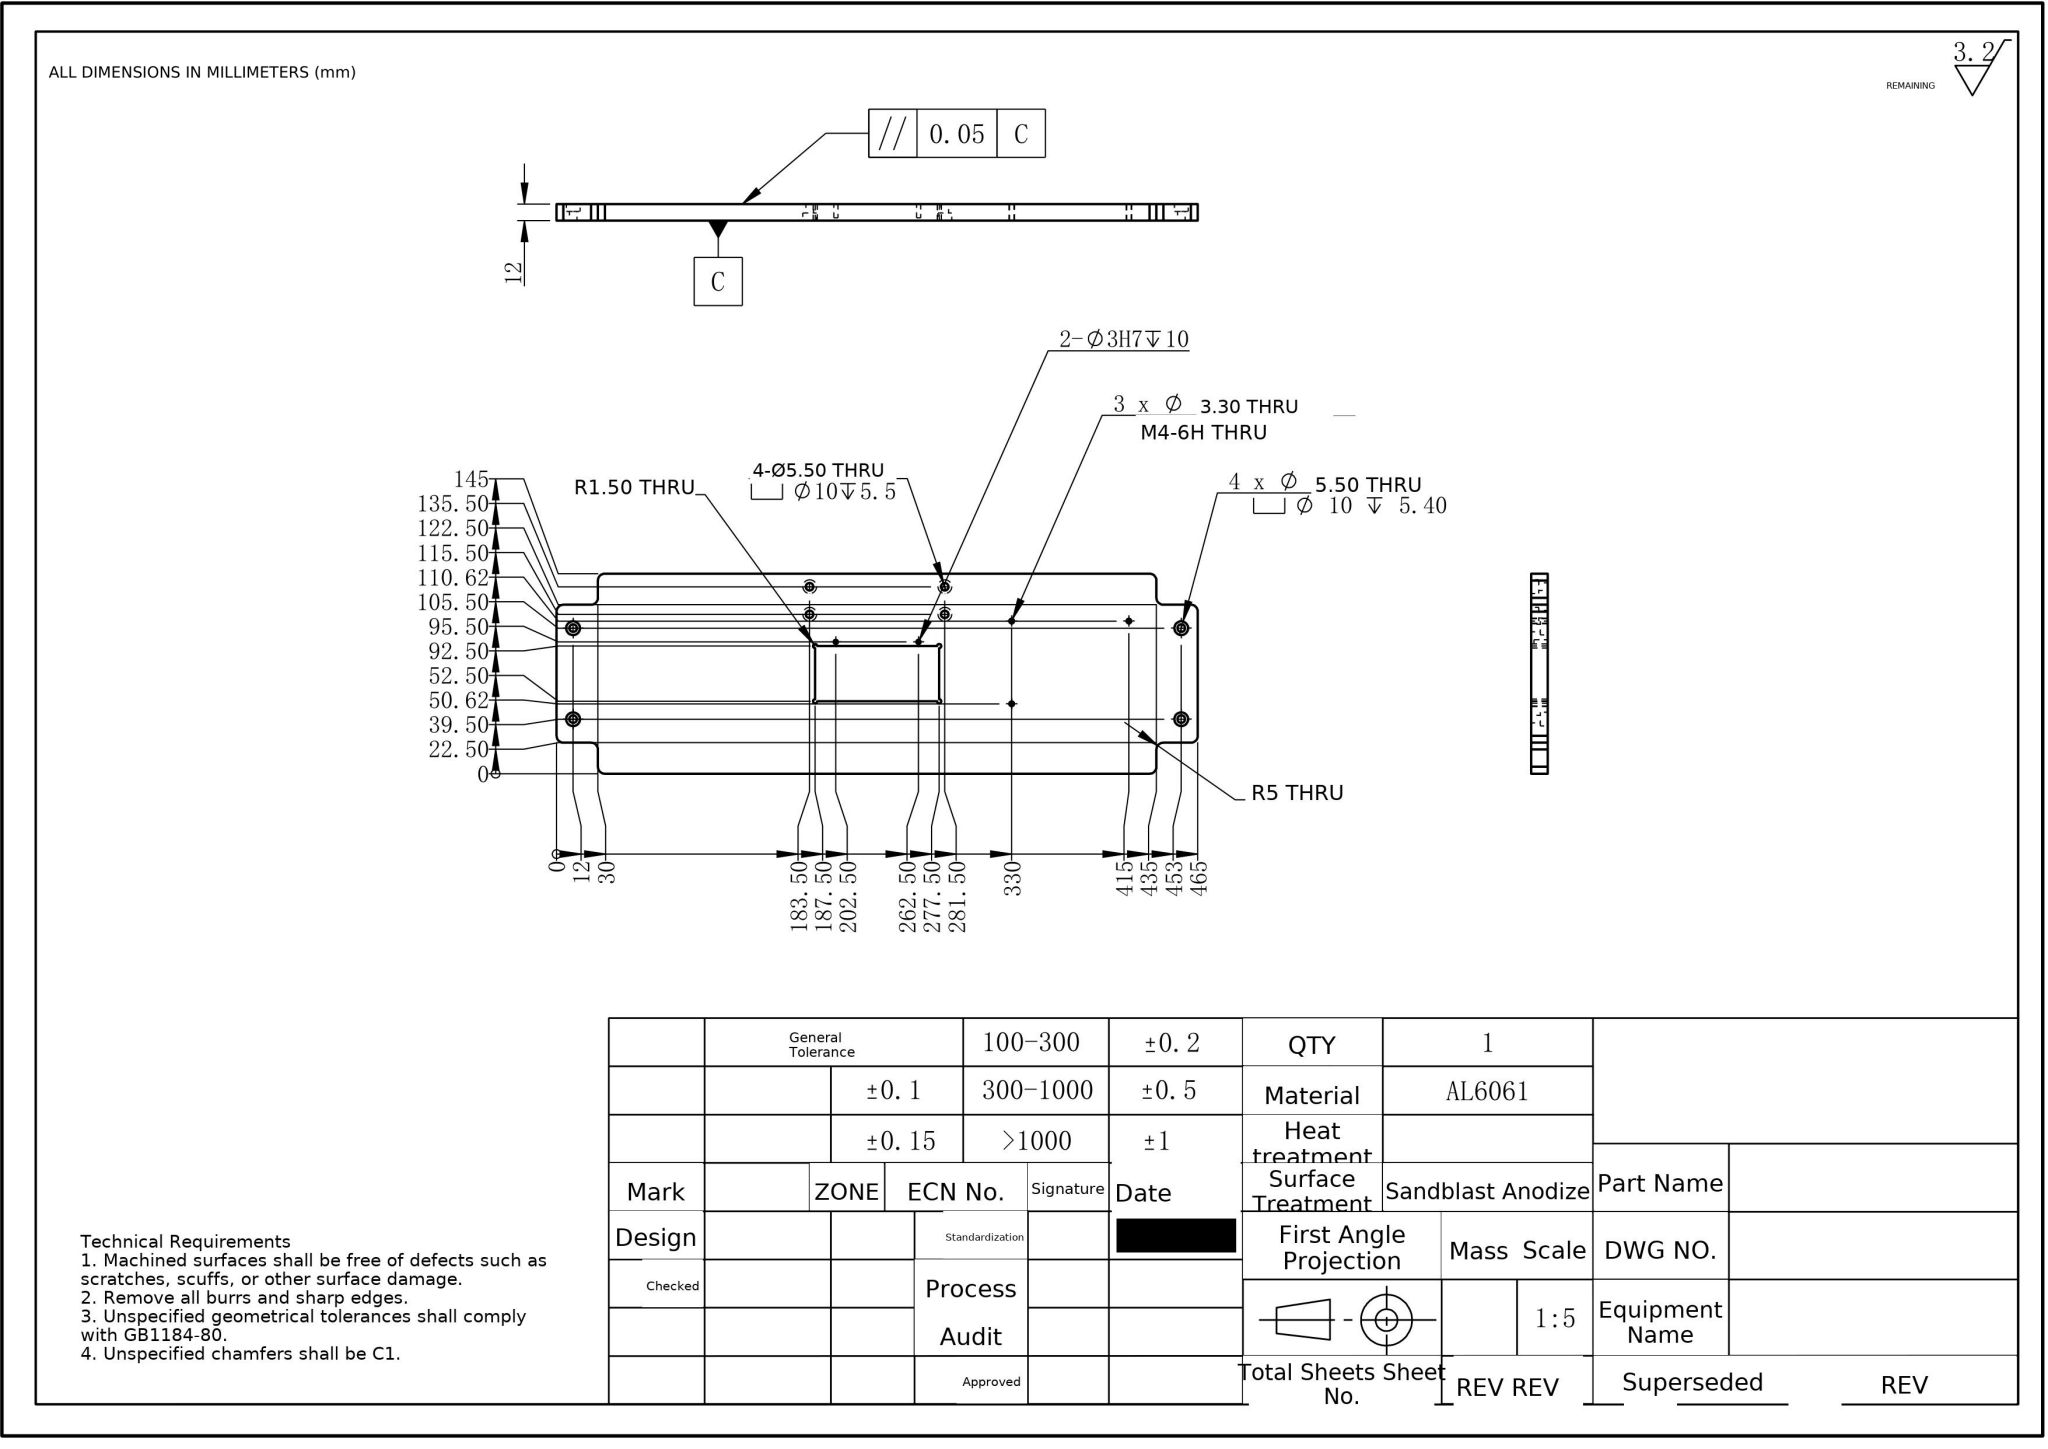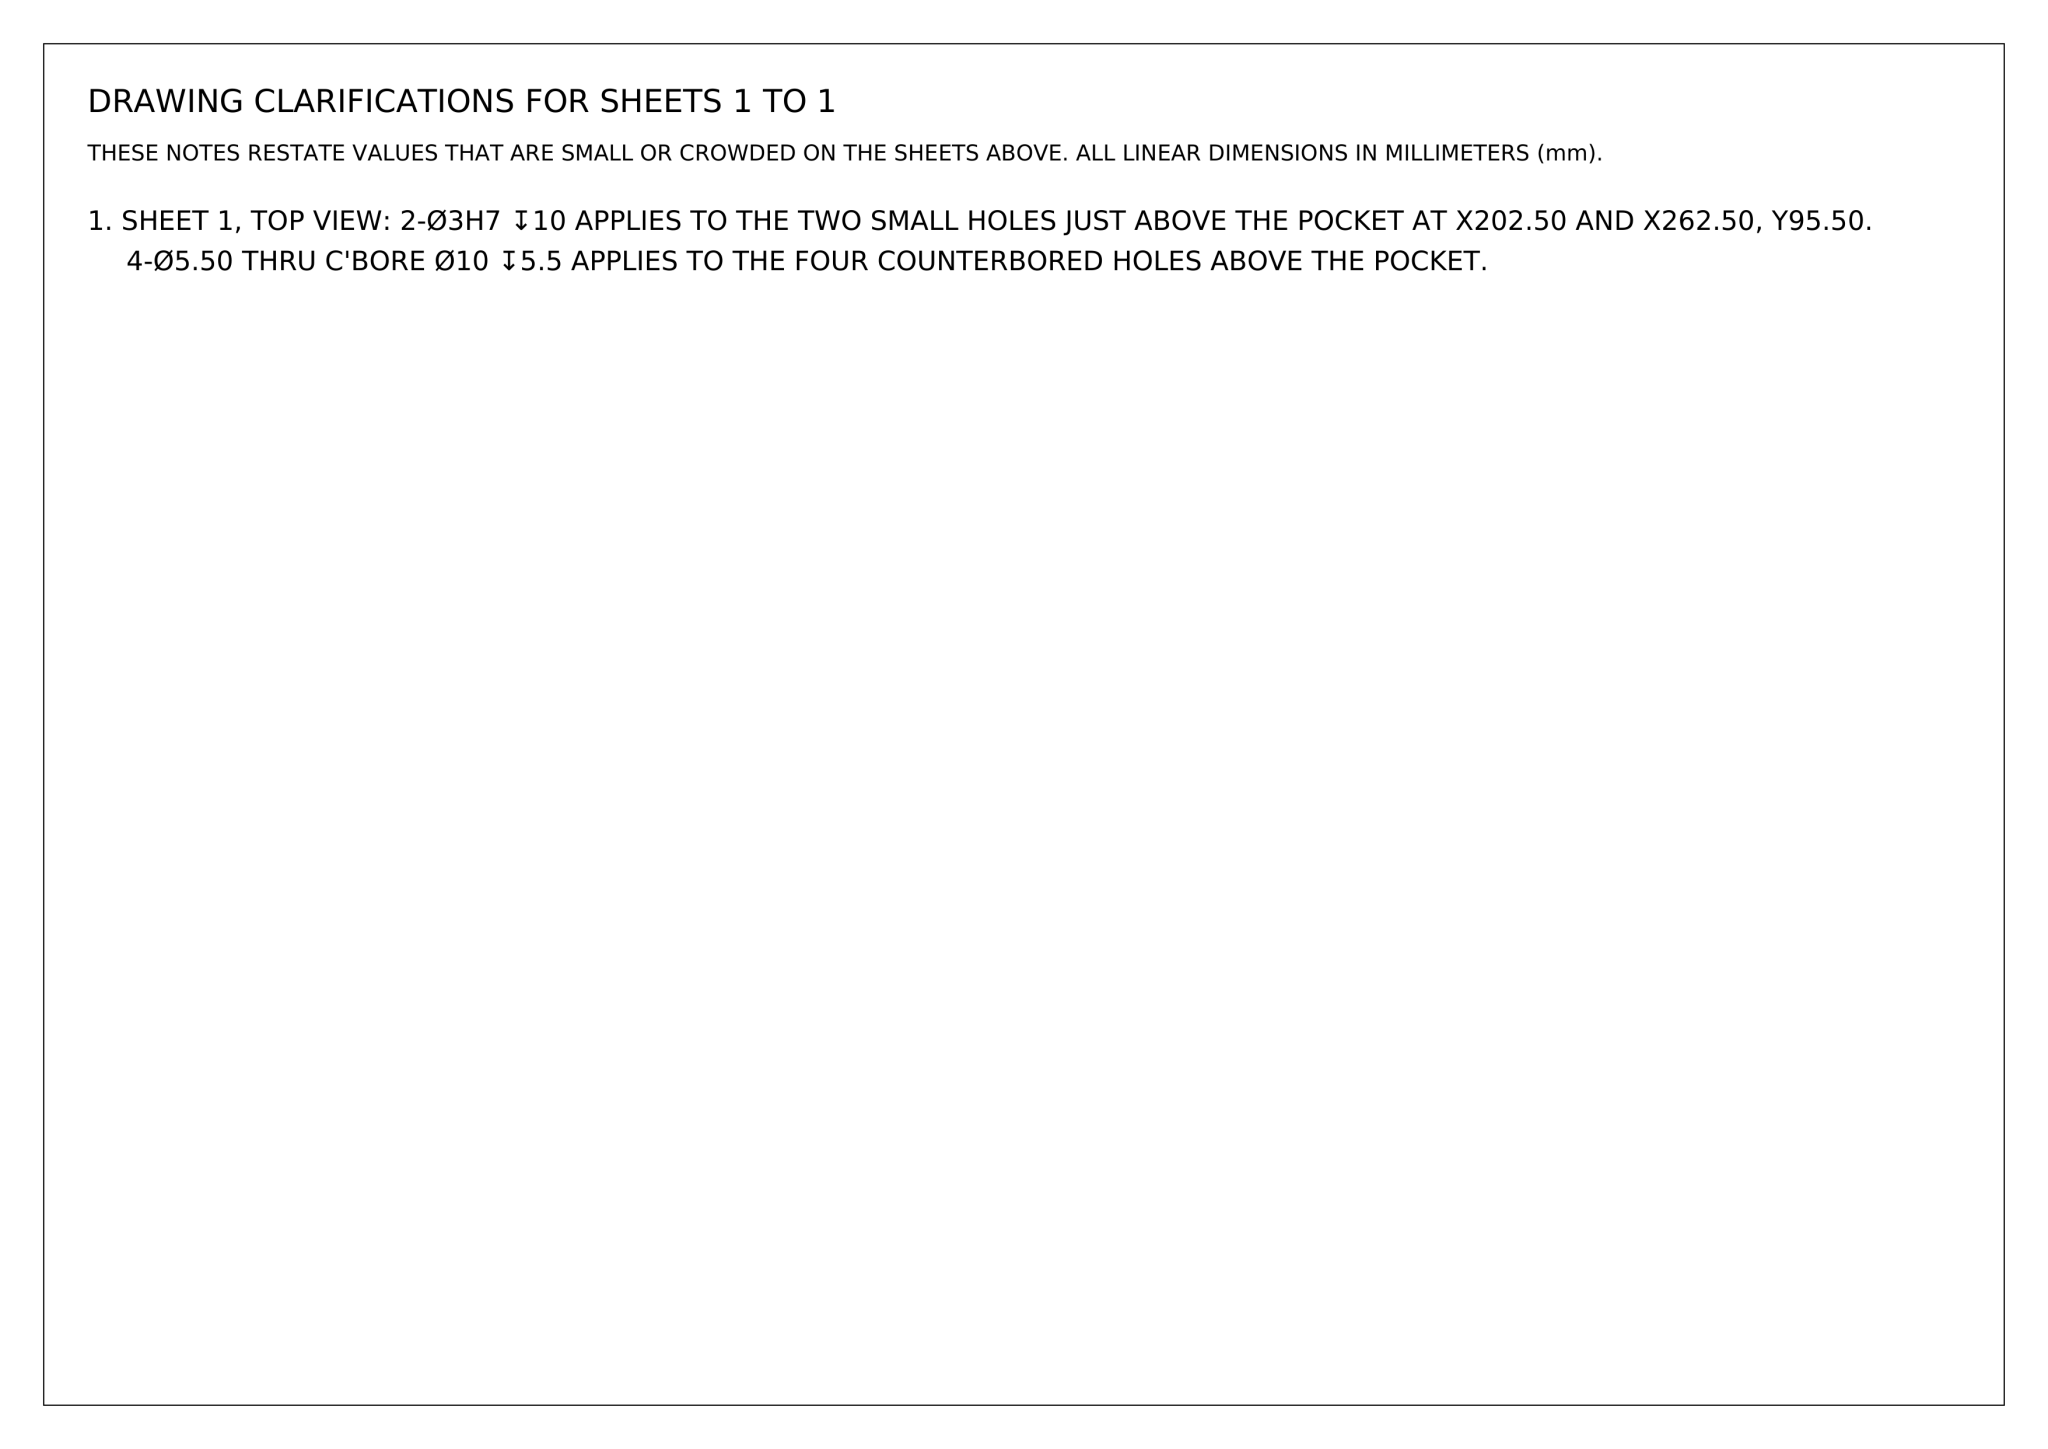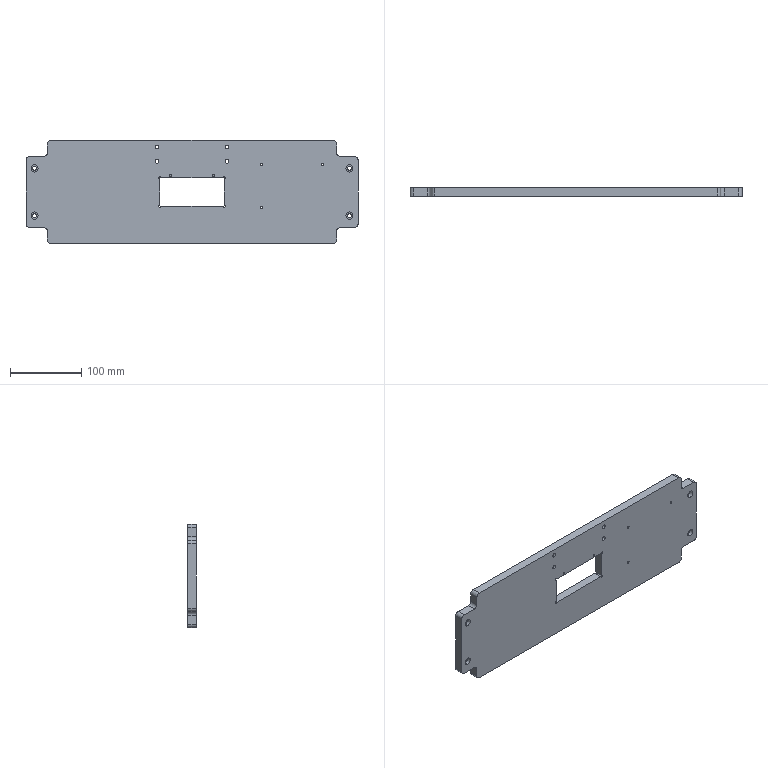Part | NX | mm | 1 solid | 88 faces | box 465 x 12 x 145 mm | volume 727869 mm3 | cylinder 60 | plane 28 | commonest cylinder face diameters 10 x28 5.5 x16 3 x10 3.3 x6